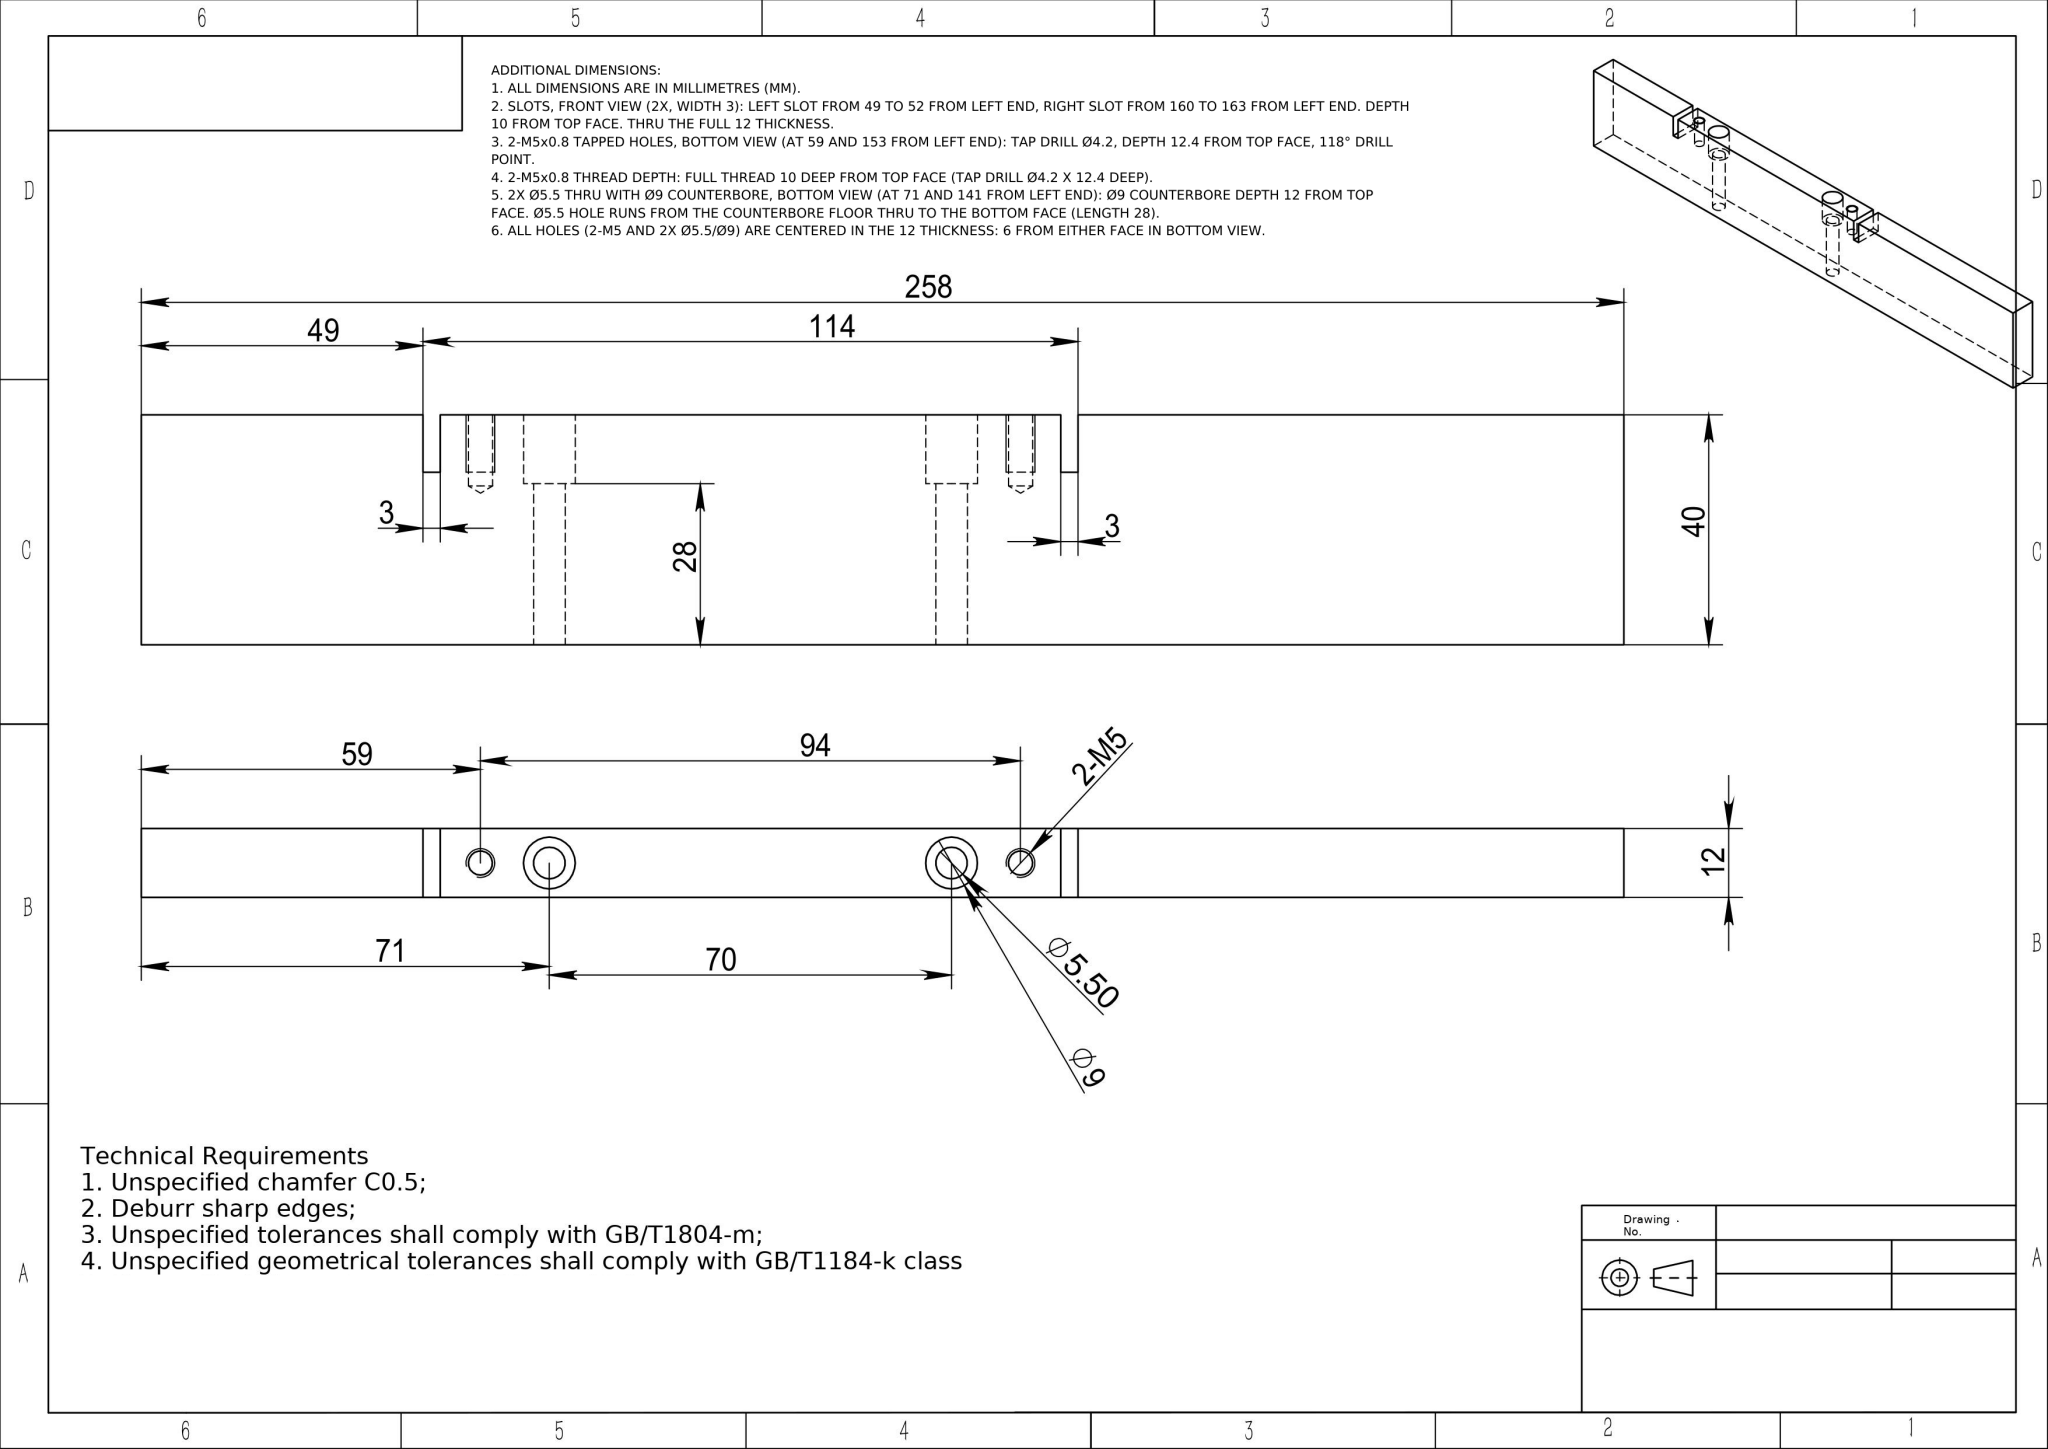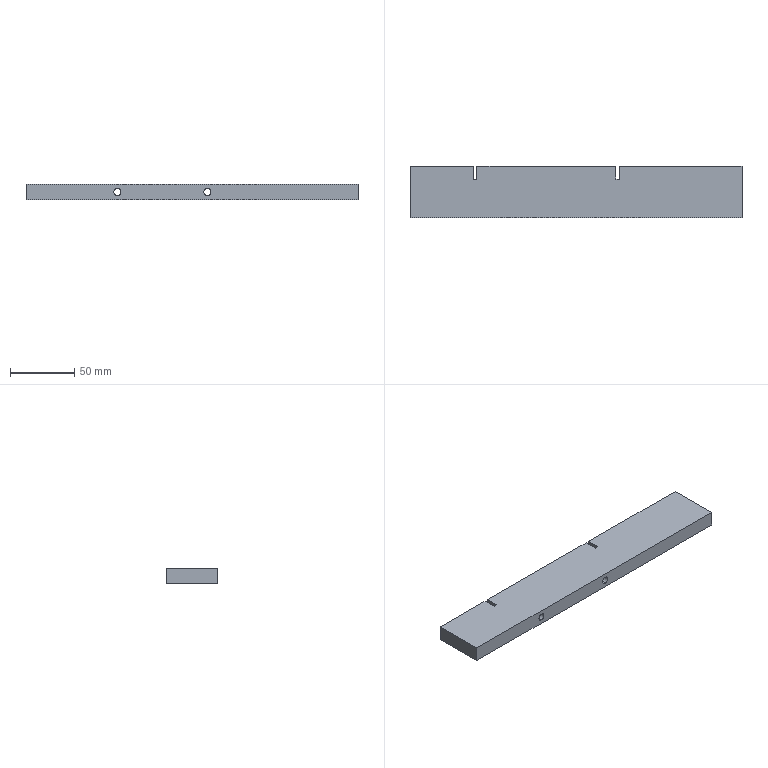Part | NX | mm | 1 solid | 32 faces | box 258 x 40 x 12 mm | volume 119907 mm3 | plane 16 | cylinder 12 | cone 4 | commonest cylinder face diameters 9 x4 4.2 x4 5.5 x4